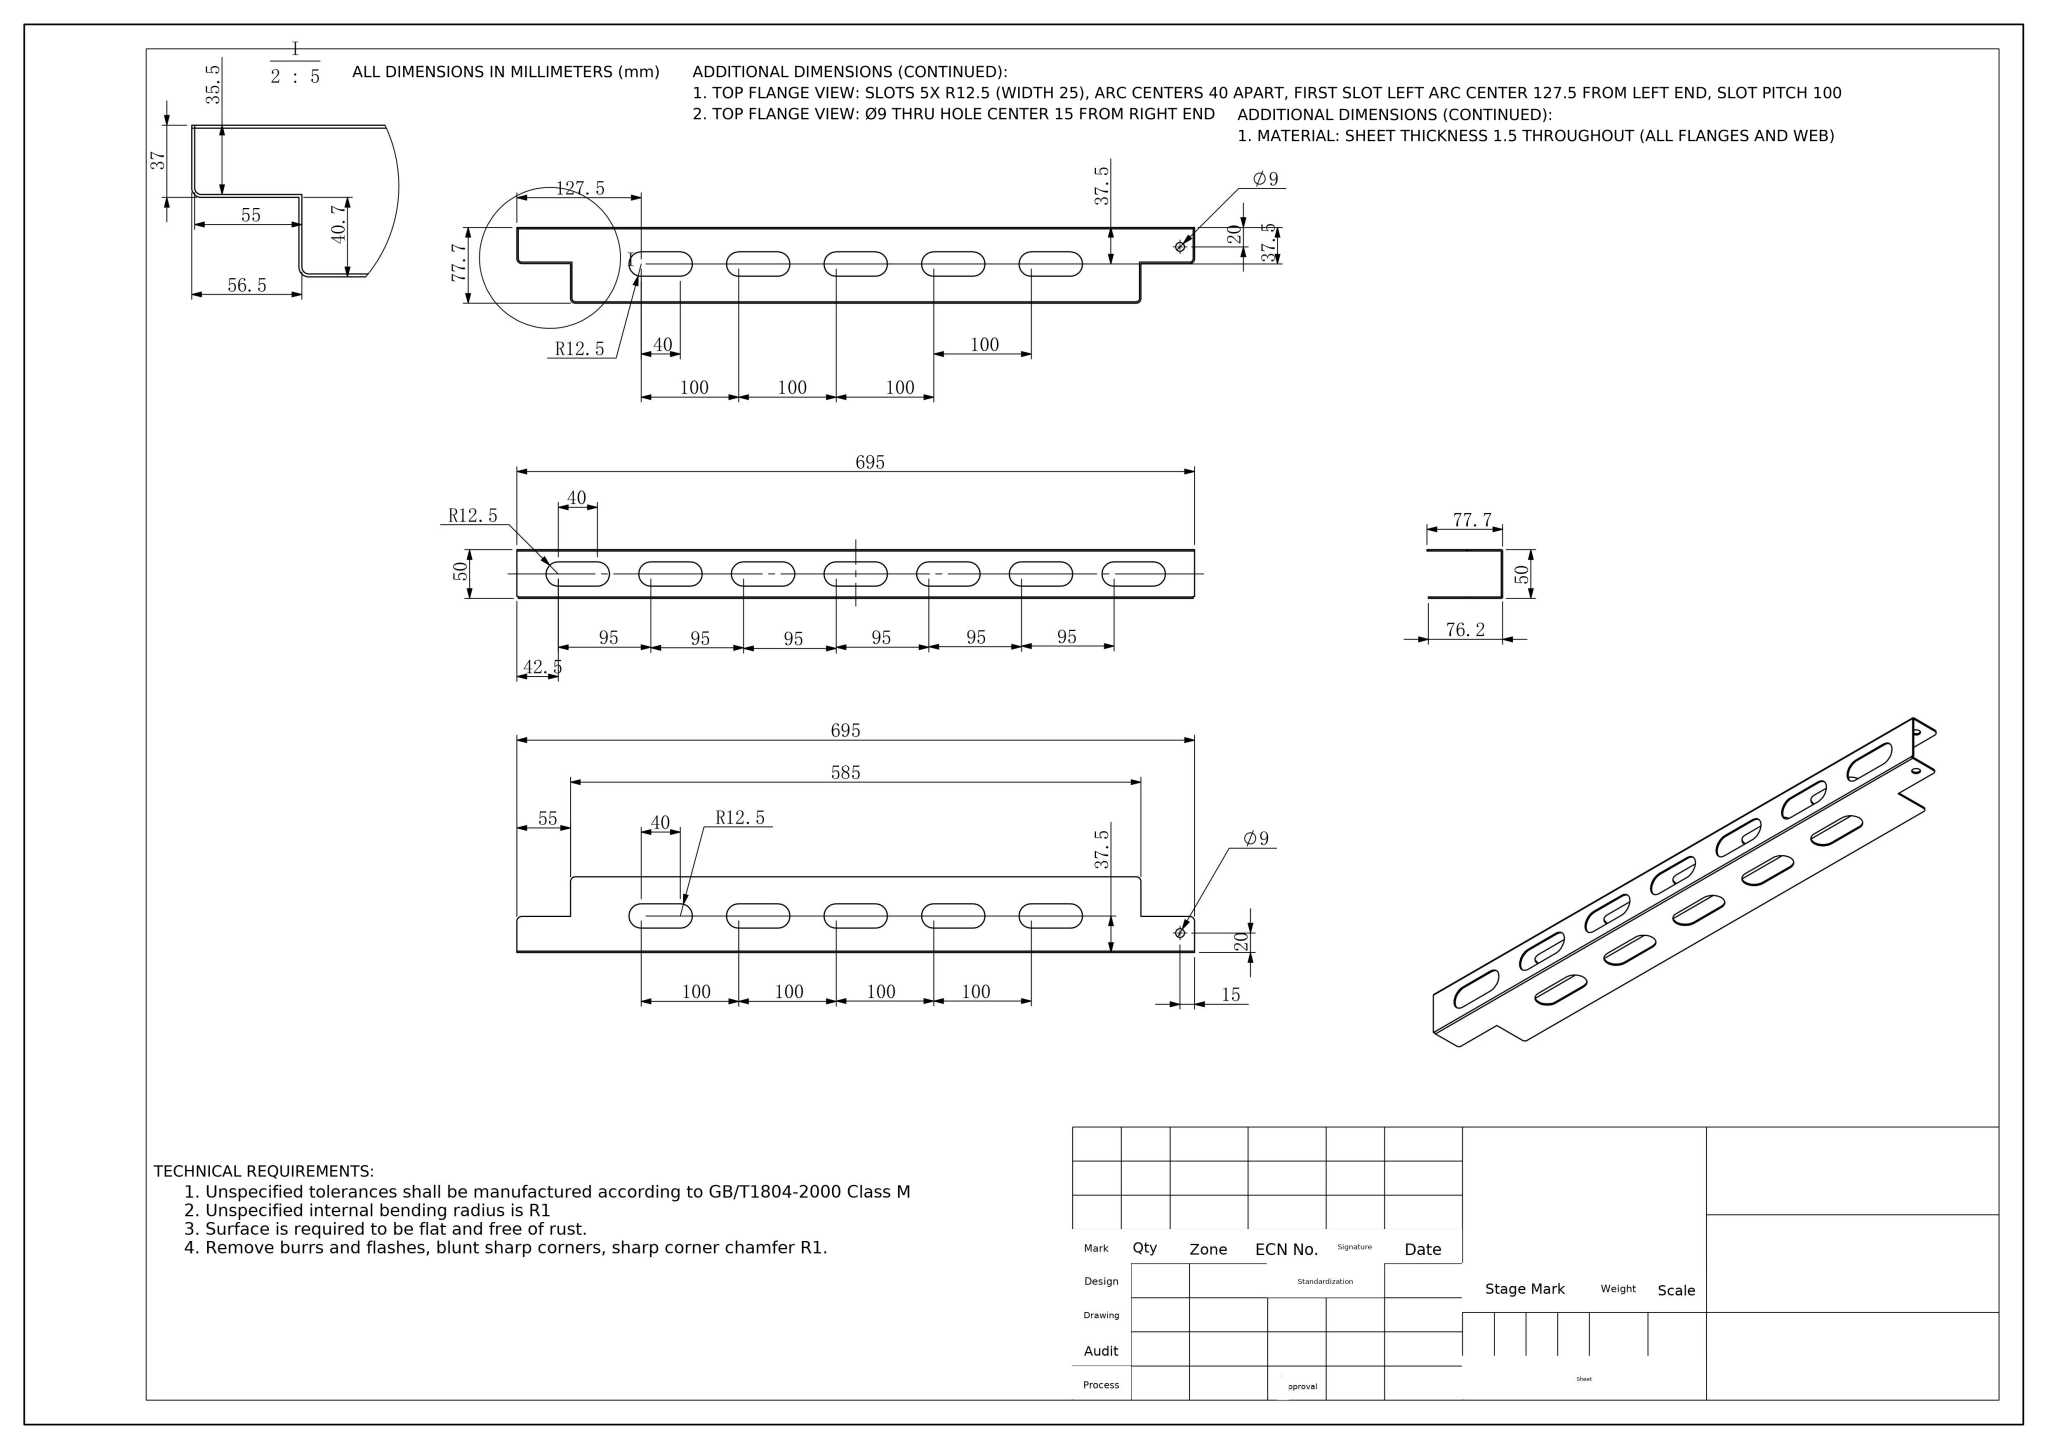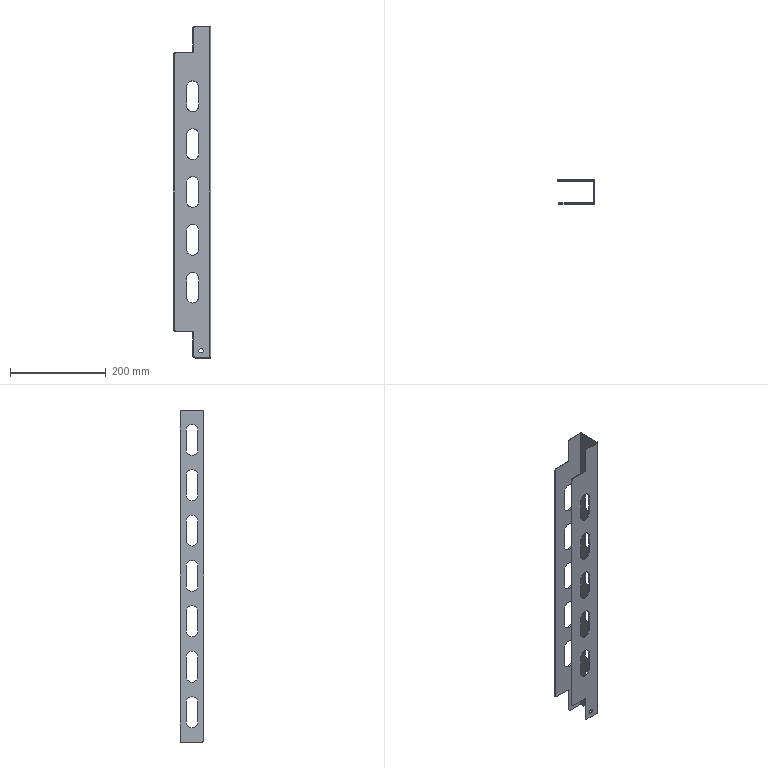Part | NX | mm | 1 solid | 131 faces | box 77.71 x 50 x 695 mm | volume 156750 mm3 | cylinder 71 | plane 60 | commonest cylinder face diameters 25 x51 10 x8 9 x4 7 x4 3.004 x2 0.004 x2